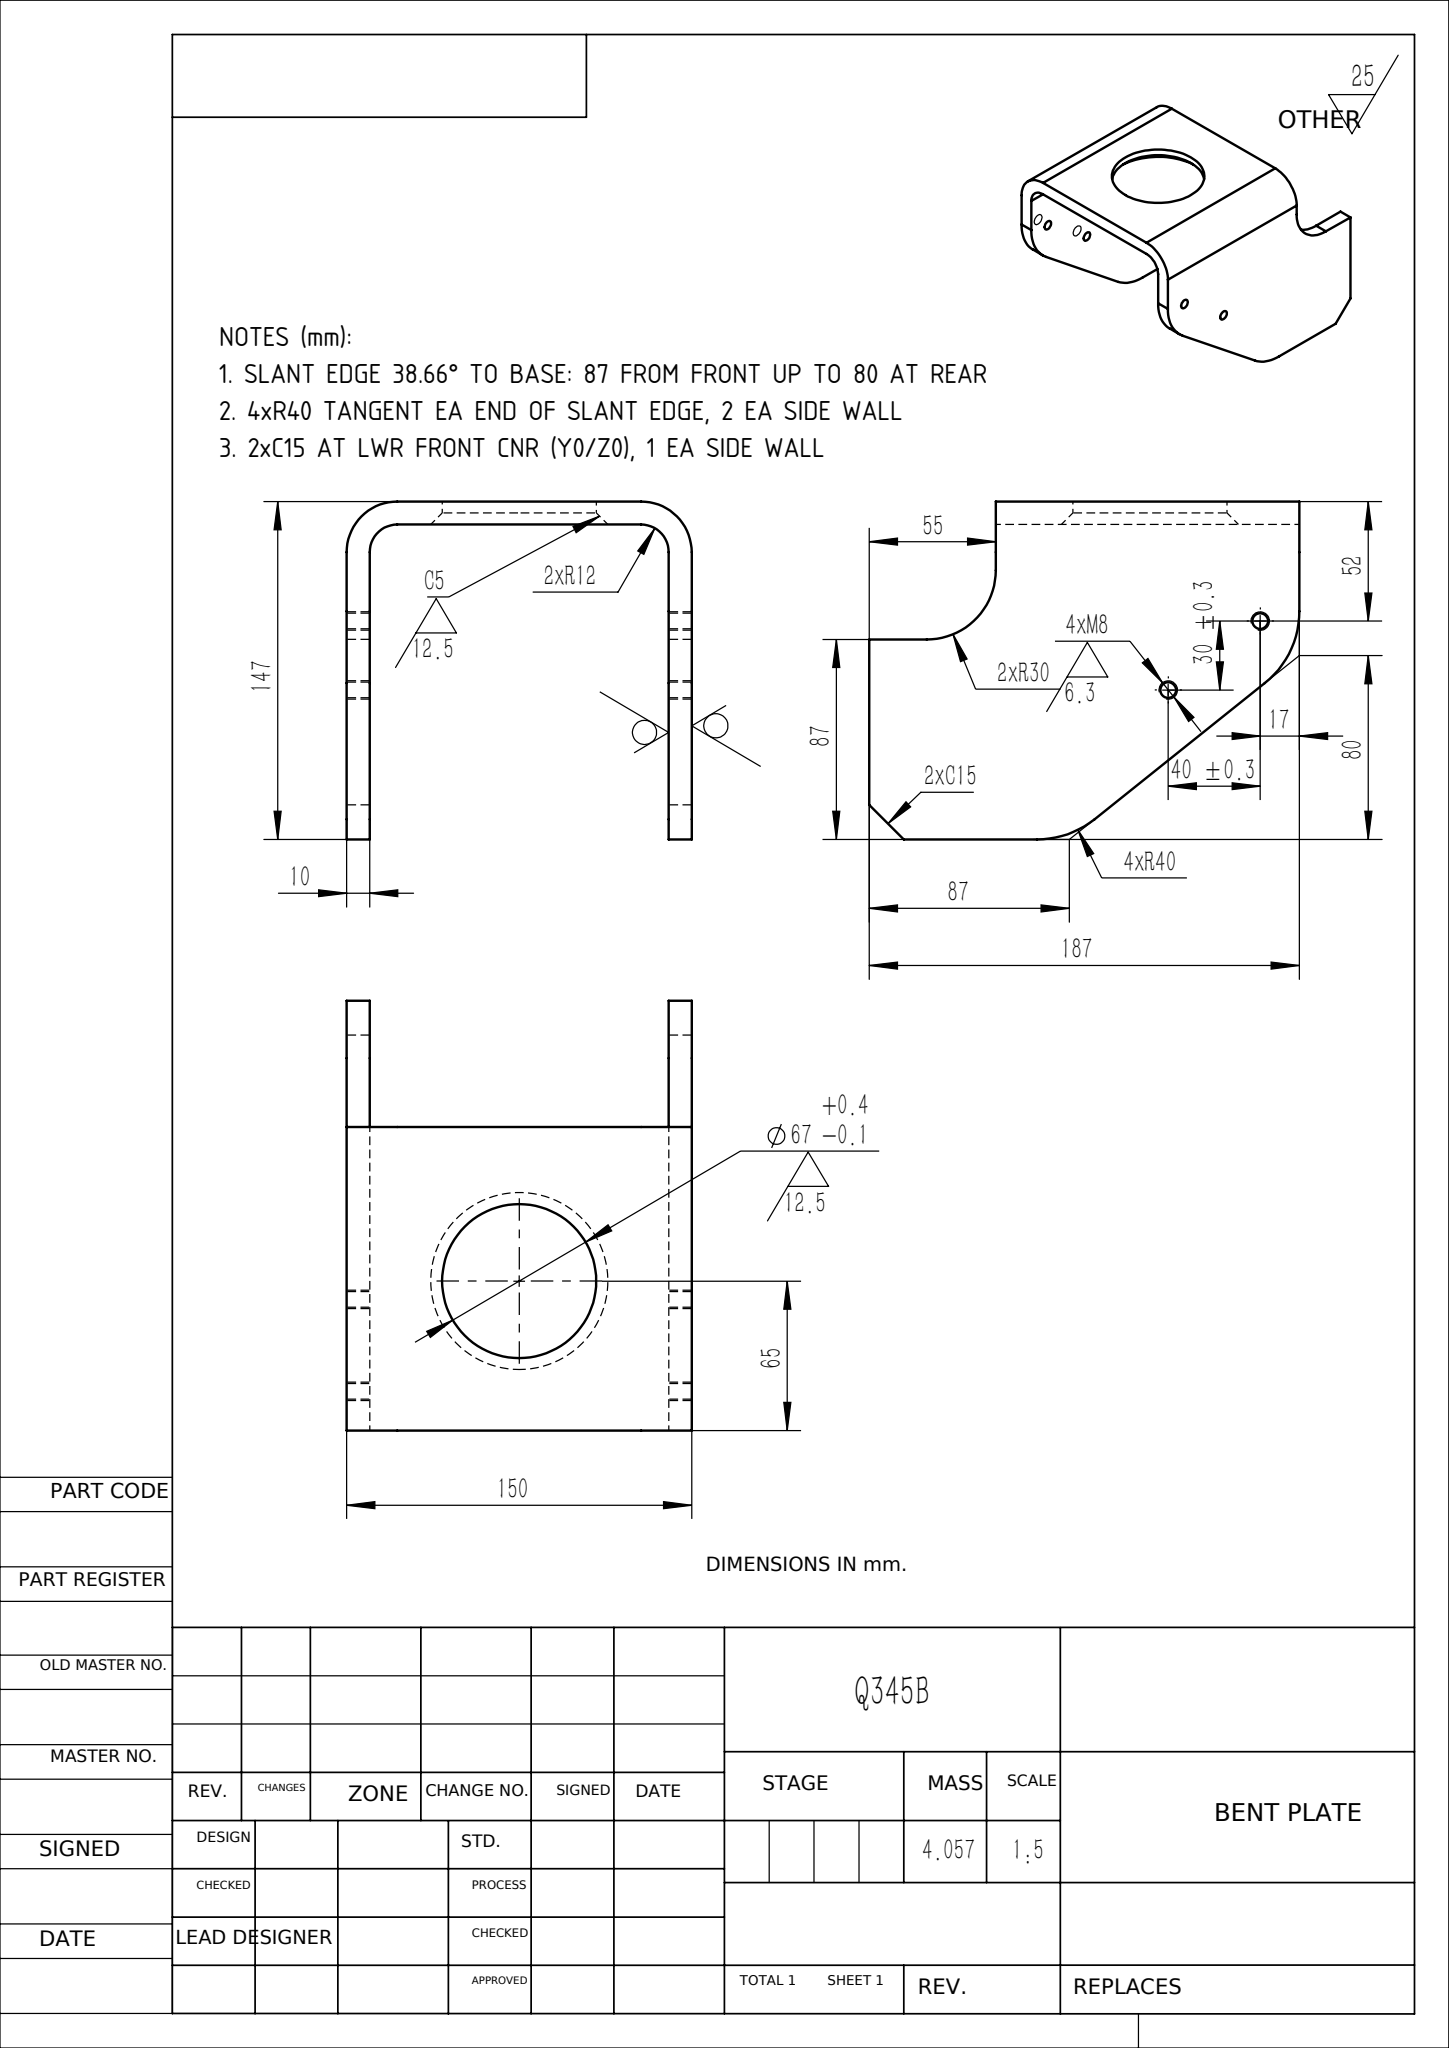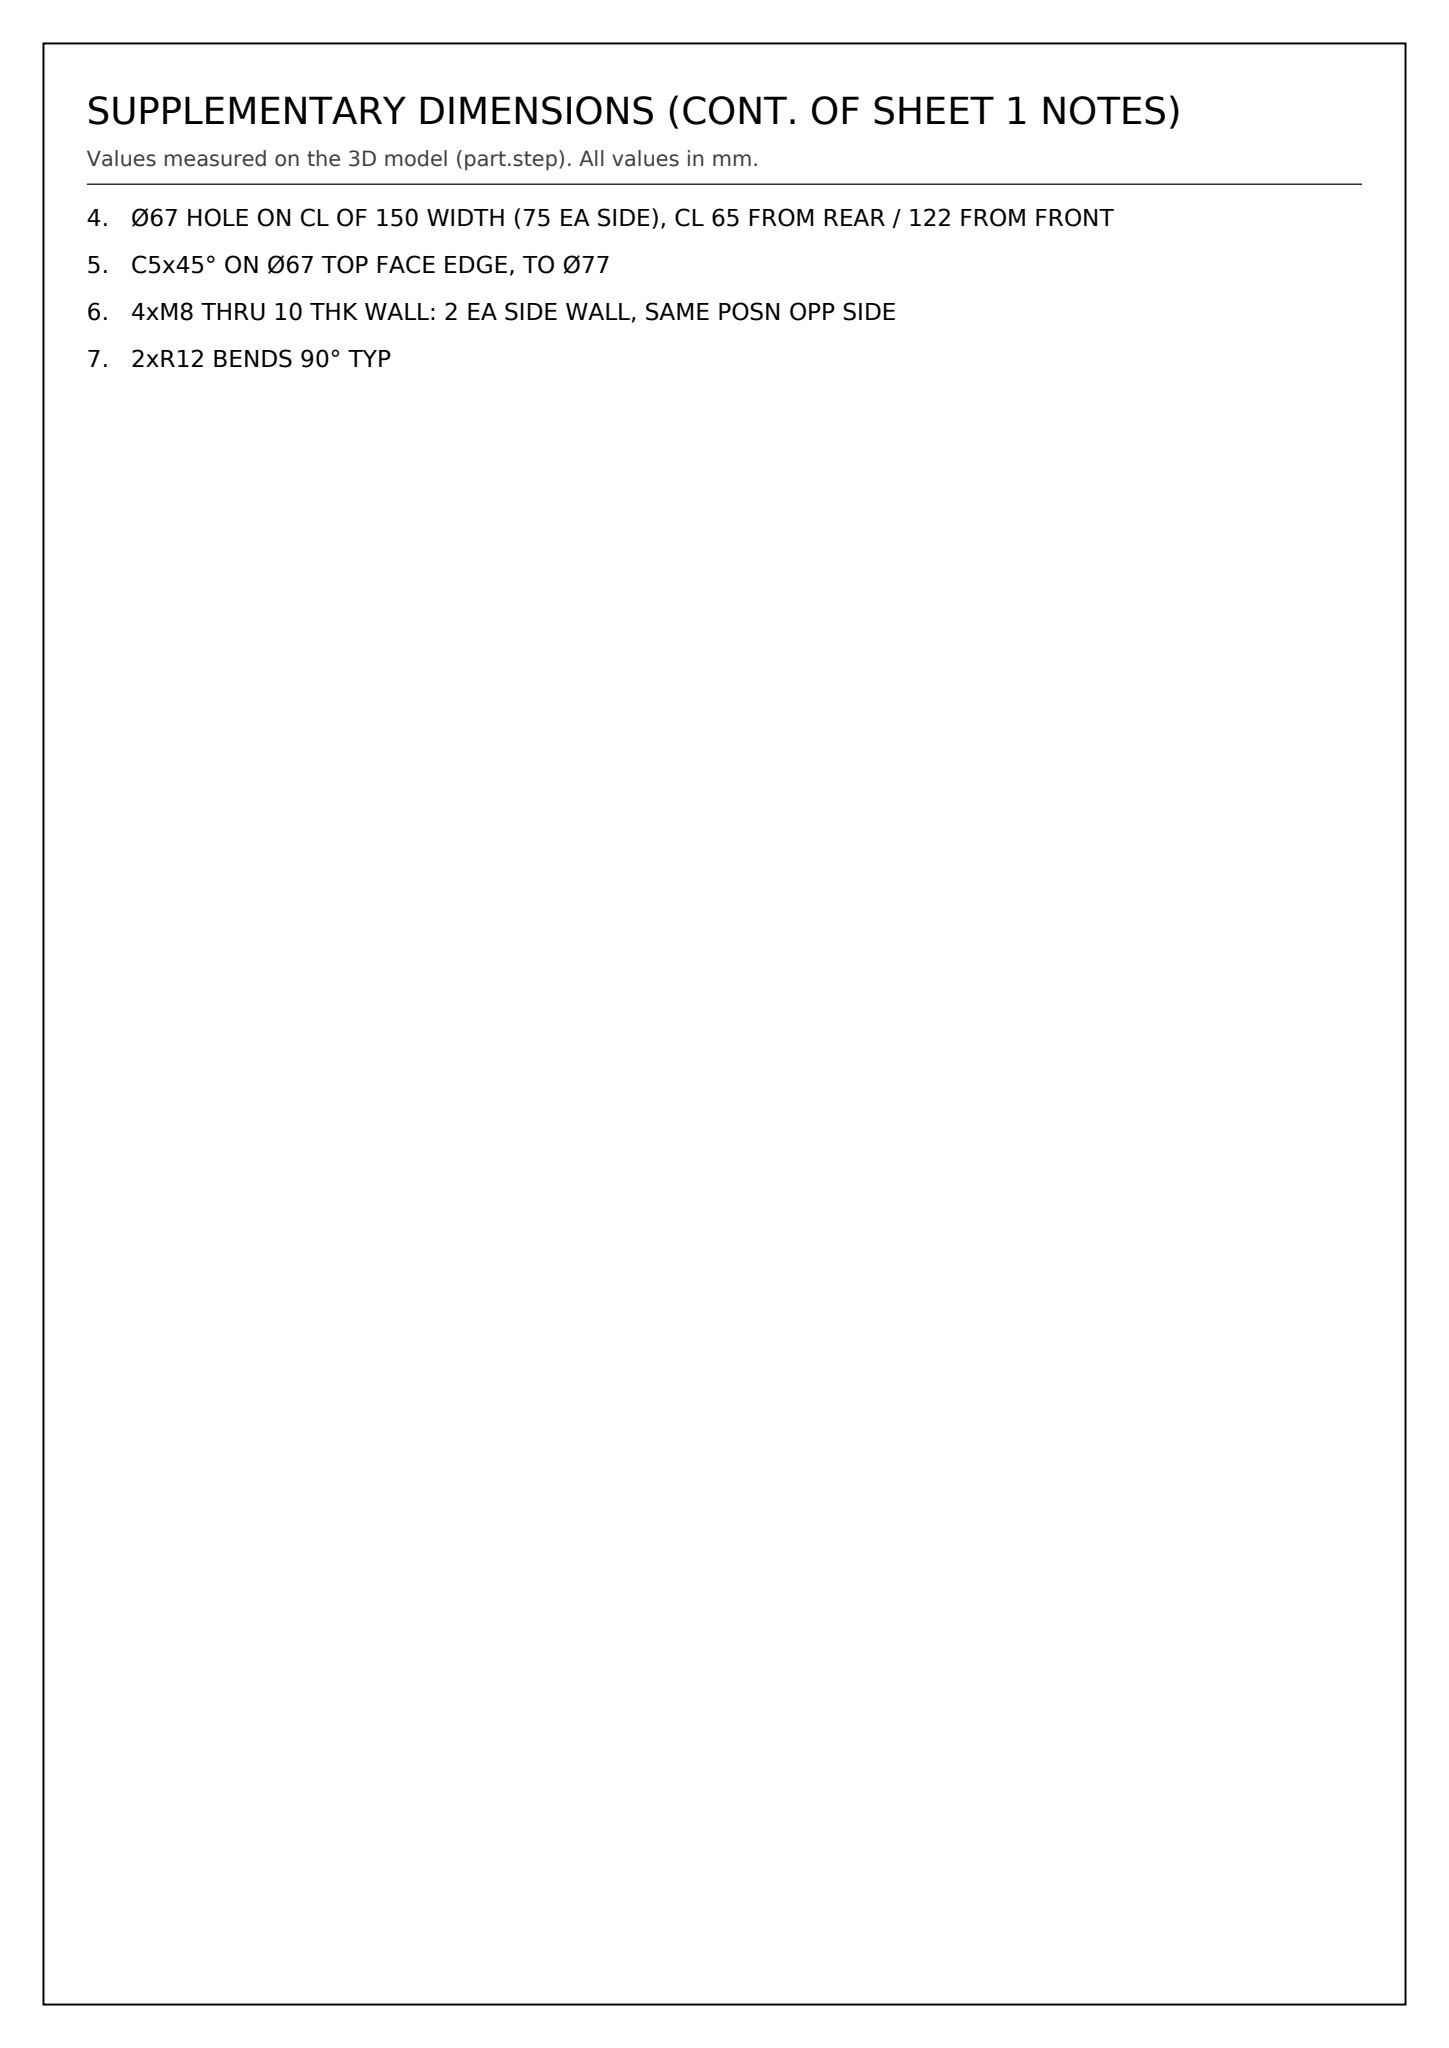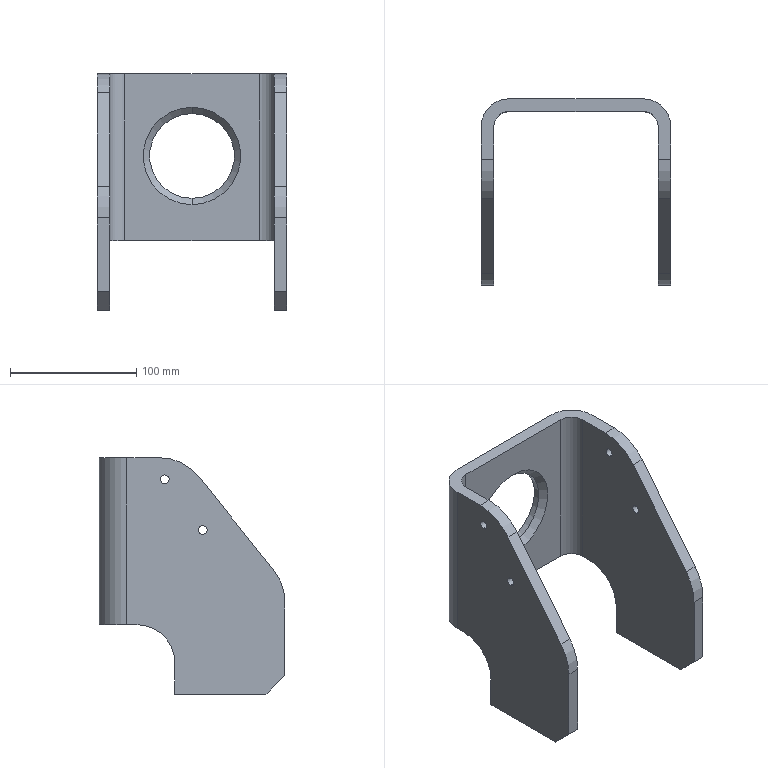Part | SolidWorks | mm | 1 solid | 40 faces | box 150 x 147 x 187 mm | volume 516787 mm3 | cylinder 20 | plane 18 | cone 2 | commonest cylinder face diameters 6.8 x8 80 x4 67 x2 60 x2 24 x2 44 x2
Drawing notes:
SLANT EDGE 38.66° TO BASE: 87 FROM FRONT UP TO 80 AT REAR | from the solid: R40 fillet ctrs (z72.97,y40) & (z147,y99.22); slope 59.22/74.03=0.800 -> 38.66°; meets y=0 at z=87, z=187 at y=80
4xR40 TANGENT EA END OF SLANT EDGE, 2 EA SIDE WALL | from the solid: Ø80 x-axis cyls at (y40,z72.97) and (y99.22,z147), len 10, 2 each = 4; tangent to y=0 and z=187
2xC15 AT LWR FRONT CNR (Y0/Z0), 1 EA SIDE WALL | from the solid: side walls at planes x0-10 & x140-150; bottom y=0, front z=0; chamfer at min corner of bbox
Ø67 HOLE ON CL OF 150 WIDTH (75 EA SIDE), CL 65 FROM REAR / 122 FROM FRONT | from the solid: Ø67 y-axis cyl at x=75, z=122; bbox x=150, z=187 -> 187-122=65 from rear
C5x45° ON Ø67 TOP FACE EDGE, TO Ø77 | from the solid: cone 90° incl, ref dia 77 coaxial with Ø67 ((77-67)/2=5)
4xM8 THRU 10 THK WALL: 2 EA SIDE WALL, SAME POSN OPP SIDE | from the solid: Ø6.8 tap-drill cyls, axis x, at (y65,z130) & (y95,z170), len 10 = wall thk (x0-10, x140-150)
2xR12 BENDS 90° TYP | from the solid: Planes x=0/10 and x=140/150 normal to y-planes 137/147; flanges perpendicular to top face
build123d program:
from build123d import *

# Parameters (mm, degrees)
BOSS_EXTRUDE1_DEPTH = 187
SKETCH2_OUTSIDE_W   = 245.242
SKETCH2_OUTSIDE_H   = 205.242
CUT_EXTRUDE1_DEPTH  = 282.208
M8_TAPPED_HOLE1_D   = 6.8
SKETCH5_R           = 33.5
CUT_EXTRUDE2_DEPTH  = 282.208
CHAMFER1_SIZE       = 5
FILLET1_R           = 12
FILLET2_R           = 22


with BuildPart() as part:
    # Sketch1 → Boss-Extrude1 (new body)
    with BuildSketch(Plane.XY):
        Polygon((0, 0), (0, 147), (150, 147), (150, 0), (140, 0), (140, 137), (10, 137), (10, 0), align=None)
    extrude(amount=BOSS_EXTRUDE1_DEPTH)

    # Sketch2 outside → Cut-Extrude1 (cut, through all)
    with BuildSketch(Plane.ZY):
        with Locations((93.5, 73.5)):
            Rectangle(SKETCH2_OUTSIDE_W, SKETCH2_OUTSIDE_H)
        with BuildLine():
            Line((187, 147), (187, 99.225))
            ThreePointArc((187, 99.225), (183.052, 81.897), (171.988, 67.99))
            Line((171.988, 67.99), (97.957, 8.765))
            ThreePointArc((97.957, 8.765), (86.209, 2.255), (72.969, 0))
            Line((72.969, 0), (15, 0))
            Line((15, 0), (0, 15))
            Line((0, 15), (0, 87))
            Line((0, 87), (25, 87))
            ThreePointArc((25, 87), (46.213, 95.787), (55, 117))
            Line((55, 117), (55, 147))
            Line((55, 147), (187, 147))
        make_face(mode=Mode.SUBTRACT)
    extrude(amount=-CUT_EXTRUDE1_DEPTH, mode=Mode.SUBTRACT)

    # M8 Tapped Hole1 (through all)
    with Locations(Plane(origin=(0, 65, 130), x_dir=(0, 0, -1), z_dir=(-1, 0, 0))):
        with Locations((0, 0), (-40, -30)):
            Hole(M8_TAPPED_HOLE1_D / 2)

    # Sketch5 → Cut-Extrude2 (cut, through all)
    with BuildSketch(Plane(origin=(0, 147, 0), x_dir=(1, 0, 0), z_dir=(0, 1, 0))):
        with Locations(Location((75, -122, 0), (0, 0, 270))):
            Circle(SKETCH5_R)
    extrude(amount=-CUT_EXTRUDE2_DEPTH, mode=Mode.SUBTRACT)

    # Chamfer1
    chamfer1_edges = [part.edges().sort_by_distance(p)[0] for p in [
        (75, 137, 88.5),
    ]]
    chamfer(chamfer1_edges, length=CHAMFER1_SIZE)

    # Fillet1
    fillet1_edges = [part.edges().sort_by_distance(p)[0] for p in [
        (140, 137, 121),
        (10, 137, 121),
    ]]
    fillet(fillet1_edges, radius=FILLET1_R)

    # Fillet2
    fillet2_edges = [part.edges().sort_by_distance(p)[0] for p in [
        (0, 147, 121),
        (150, 147, 121),
    ]]
    fillet(fillet2_edges, radius=FILLET2_R)


solid = part.part